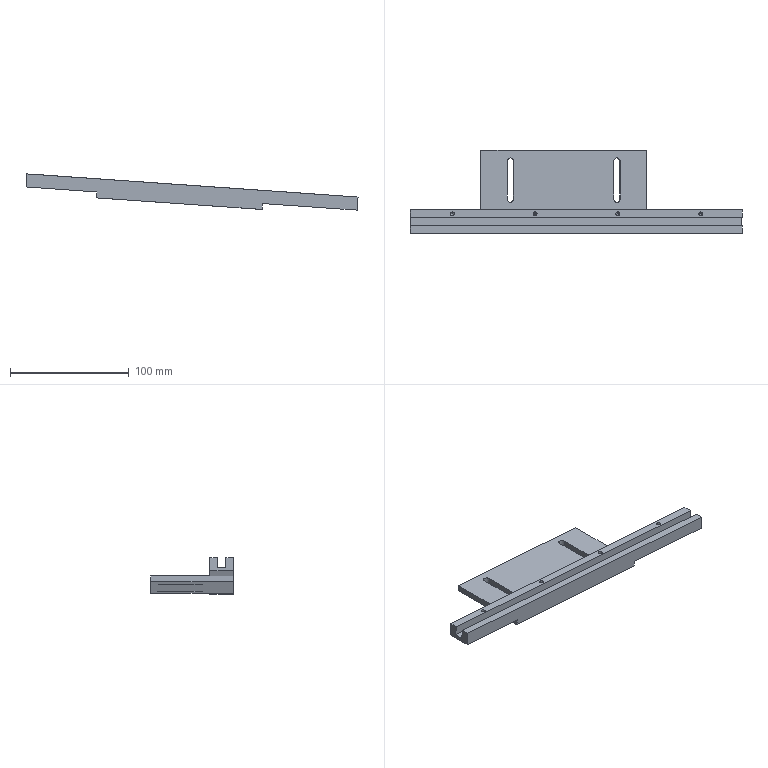Component | SolidWorks | CSFA2082 079-1 | 1 solid | 40 faces | box 280.09 x 70 x 30.6 mm | volume 92703 mm3 | plane 20 | cylinder 12 | cone 8 | commonest cylinder face diameters 3.3 x8 5.5 x4
build123d program:
from build123d import *

# Parameters (mm, degrees)
SKETCH1_W                 = 140
SKETCH1_H                 = 70
EXTRUDE1_DEPTH            = 5
SKETCH2_W                 = 220
SKETCH2_H                 = 20
EXTRUDE2_DEPTH            = 14
SKETCH3_W                 = 60
SKETCH3_H                 = 20
EXTRUDE3_DEPTH            = 14
SKETCH4_W                 = 8.2
SKETCH4_H                 = 7.1
CUT_EXTRUDE1_DEPTH        = 283.818
SKETCH5_R                 = 2.75
CUT_EXTRUDE2_DEPTH        = 155.664
CUT_EXTRUDE3_DEPTH        = 155.664
SKETCH7_W                 = 2.9
SKETCH7_H                 = 20
CUT_EXTRUDE4_DEPTH        = 283.818
M4X0_7_TAPPED_HOLE1_D     = 3.3
M4X0_7_TAPPED_HOLE1_DEPTH = 10.1
M4X0_7_TAPPED_HOLE1_TIP   = 0.9914


with BuildPart() as part:
    # Sketch1 → Extrude1 (new body)
    with BuildSketch(Plane.XY):
        Rectangle(SKETCH1_W, SKETCH1_H)
    extrude(amount=EXTRUDE1_DEPTH)

    # Sketch2 → Extrude2 (add)
    with BuildSketch(Plane.XY.offset(5)):
        with Locations((-40, 25)):
            Rectangle(SKETCH2_W, SKETCH2_H)
    extrude(amount=EXTRUDE2_DEPTH)

    # Sketch3 → Extrude3 (add)
    with BuildSketch(Plane.XY.offset(5)):
        with Locations((100, 25)):
            Rectangle(SKETCH3_W, SKETCH3_H)
    extrude(amount=EXTRUDE3_DEPTH)

    # Sketch4 → Cut-Extrude1 (cut, through all)
    with BuildSketch(Plane(origin=(130, 0, 0), x_dir=(0, 0, -1), z_dir=(1, 0, 0))):
        with Locations((-12.1, 25)):
            Rectangle(SKETCH4_W, SKETCH4_H)
    extrude(amount=-CUT_EXTRUDE1_DEPTH, mode=Mode.SUBTRACT)

    # Sketch5 → Cut-Extrude2 (cut, through all)
    with BuildSketch(Plane.XY.offset(5)):
        with Locations((-45, 6)):
            Circle(SKETCH5_R)
        with Locations(Location((45, 6, 0), (0, 0, 180))):
            Circle(SKETCH5_R)
        with Locations((45, -26)):
            Circle(SKETCH5_R)
        with Locations(Location((-45, -26, 0), (0, 0, 180))):
            Circle(SKETCH5_R)
    extrude(amount=-CUT_EXTRUDE2_DEPTH, mode=Mode.SUBTRACT)

    # Sketch6 → Cut-Extrude3 (cut, through all)
    with BuildSketch(Plane.XY.offset(5)):
        with BuildLine():
            Line((-42.25, 6), (-42.25, -26))
            ThreePointArc((-42.25, -26), (-45, -28.75), (-47.75, -26))
            Line((-47.75, -26), (-47.75, 6))
            ThreePointArc((-47.75, 6), (-45, 8.75), (-42.25, 6))
        make_face()
        with BuildLine():
            Line((47.75, 6), (47.75, -26))
            ThreePointArc((47.75, -26), (45, -28.75), (42.25, -26))
            Line((42.25, -26), (42.25, 6))
            ThreePointArc((42.25, 6), (45, 8.75), (47.75, 6))
        make_face()
    extrude(amount=-CUT_EXTRUDE3_DEPTH, mode=Mode.SUBTRACT)

    # Sketch7 → Cut-Extrude4 (cut, through all)
    with BuildSketch(Plane(origin=(130, 0, 0), x_dir=(0, 0, -1), z_dir=(1, 0, 0))):
        with Locations((-17.55, 25)):
            Rectangle(SKETCH7_W, SKETCH7_H)
    extrude(amount=-CUT_EXTRUDE4_DEPTH, mode=Mode.SUBTRACT)

    # M4x0.7 Tapped Hole1
    with Locations(Plane.XY.offset(16.1)):
        with Locations((95, 18.5), (25, 18.5), (-45, 18.5), (-115, 18.5)):
            Hole(M4X0_7_TAPPED_HOLE1_D / 2, depth=M4X0_7_TAPPED_HOLE1_DEPTH)
            with Locations((0, 0, -(M4X0_7_TAPPED_HOLE1_DEPTH + M4X0_7_TAPPED_HOLE1_TIP / 2))):  # 118° drill point
                Cone(0, M4X0_7_TAPPED_HOLE1_D / 2, M4X0_7_TAPPED_HOLE1_TIP, mode=Mode.SUBTRACT)


solid = part.part

# Placed as in the assembly
solid = solid.moved(Location((178.765, -218.176, 786.093), (0, 4, 180)))